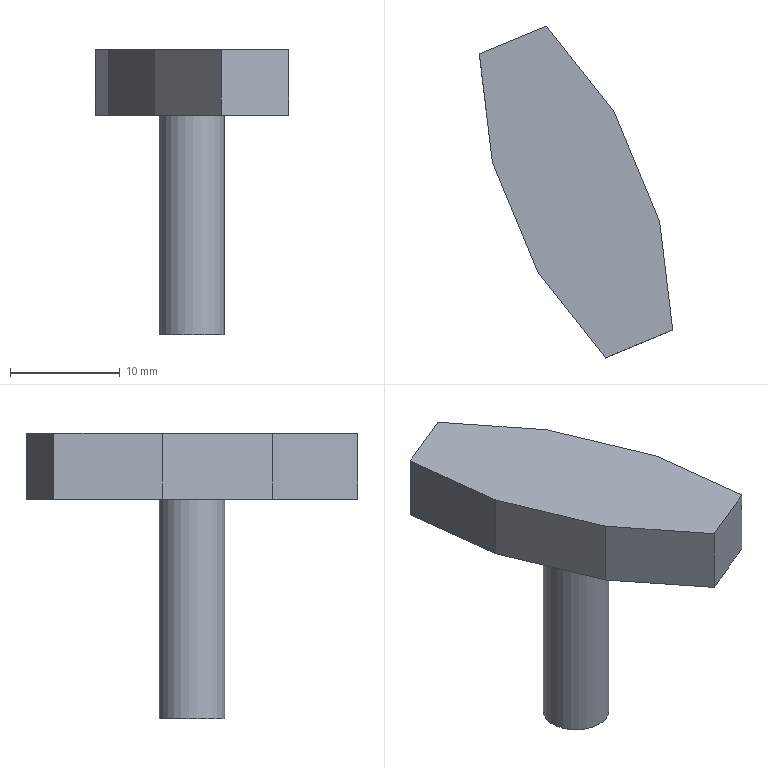Component | NX | MANUAL_SCREW | 1 solid | 12 faces | box 17.62 x 30.25 x 26 mm | volume 2418 mm3 | plane 11 | cylinder 1 | commonest cylinder face diameters 6 x1
STEP:
#1=CARTESIAN_POINT('',(0.,0.,0.));
#2=DIRECTION('',(0.,0.,1.));
#3=DIRECTION('',(1.,0.,0.));
#4=AXIS2_PLACEMENT_3D('',#1,#2,#3);
#5=CARTESIAN_POINT('',(97.911,100.613,38.296));
#6=VERTEX_POINT('',#5);
#7=CARTESIAN_POINT('',(96.724,110.478,38.296));
#8=VERTEX_POINT('',#7);
#9=CARTESIAN_POINT('',(97.911,100.613,38.296));
#10=DIRECTION('',(-0.1195,0.9928,0.));
#11=VECTOR('',#10,1.);
#12=LINE('',#9,#11);
#13=CARTESIAN_POINT('',(97.911,100.613,32.296));
#14=DIRECTION('',(0.9928,0.1195,0.));
#15=DIRECTION('',(0.1195,-0.9928,0.));
#16=AXIS2_PLACEMENT_3D('',#13,#14,#15);
#17=PLANE('',#16);
#18=CARTESIAN_POINT('',(0.,-6.));
#19=DIRECTION('',(-1.,0.));
#20=VECTOR('',#19,1.);
#21=LINE('',#18,#20);
#22=(GEOMETRIC_REPRESENTATION_CONTEXT(2)PARAMETRIC_REPRESENTATION_CONTEXT()REPRESENTATION_CONTEXT('',''));
#23=DEFINITIONAL_REPRESENTATION('',(#21),#22);
#24=PCURVE('',#17,#23);
#25=CARTESIAN_POINT('',(105.534,97.893,38.296));
#26=DIRECTION('',(0.,0.,-1.));
#27=DIRECTION('',(0.9237,0.383,0.));
#28=AXIS2_PLACEMENT_3D('',#25,#26,#27);
#29=PLANE('',#28);
#30=CARTESIAN_POINT('',(-6.,-5.433));
#31=DIRECTION('',(0.2699,-0.9629));
#32=VECTOR('',#31,1.);
#33=LINE('',#30,#32);
#34=(GEOMETRIC_REPRESENTATION_CONTEXT(2)PARAMETRIC_REPRESENTATION_CONTEXT()REPRESENTATION_CONTEXT('',''));
#35=DEFINITIONAL_REPRESENTATION('',(#33),#34);
#36=PCURVE('',#29,#35);
#37=SURFACE_CURVE('',#12,(#24,#36),.PCURVE_S1.);
#38=EDGE_CURVE('',#6,#8,#37,.T.);
#39=ORIENTED_EDGE('',*,*,#38,.T.);
#40=CARTESIAN_POINT('',(96.724,110.478,32.296));
#41=VERTEX_POINT('',#40);
#42=CARTESIAN_POINT('',(96.724,110.478,32.296));
#43=DIRECTION('',(0.,0.,1.));
#44=VECTOR('',#43,1.);
#45=LINE('',#42,#44);
#46=CARTESIAN_POINT('',(-9.936,0.));
#47=DIRECTION('',(0.,-1.));
#48=VECTOR('',#47,1.);
#49=LINE('',#46,#48);
#50=(GEOMETRIC_REPRESENTATION_CONTEXT(2)PARAMETRIC_REPRESENTATION_CONTEXT()REPRESENTATION_CONTEXT('',''));
#51=DEFINITIONAL_REPRESENTATION('',(#49),#50);
#52=PCURVE('',#17,#51);
#53=CARTESIAN_POINT('',(99.789,111.749,32.296));
#54=DIRECTION('',(0.383,-0.9237,0.));
#55=DIRECTION('',(0.,0.,-1.));
#56=AXIS2_PLACEMENT_3D('',#53,#54,#55);
#57=PLANE('',#56);
#58=CARTESIAN_POINT('',(0.,-3.318));
#59=DIRECTION('',(-1.,0.));
#60=VECTOR('',#59,1.);
#61=LINE('',#58,#60);
#62=(GEOMETRIC_REPRESENTATION_CONTEXT(2)PARAMETRIC_REPRESENTATION_CONTEXT()REPRESENTATION_CONTEXT('',''));
#63=DEFINITIONAL_REPRESENTATION('',(#61),#62);
#64=PCURVE('',#57,#63);
#65=SURFACE_CURVE('',#45,(#52,#64),.PCURVE_S1.);
#66=EDGE_CURVE('',#41,#8,#65,.T.);
#67=ORIENTED_EDGE('',*,*,#66,.F.);
#68=CARTESIAN_POINT('',(97.911,100.613,32.296));
#69=VERTEX_POINT('',#68);
#70=CARTESIAN_POINT('',(97.911,100.613,32.296));
#71=DIRECTION('',(-0.1195,0.9928,0.));
#72=VECTOR('',#71,1.);
#73=LINE('',#70,#72);
#74=CARTESIAN_POINT('',(0.,0.));
#75=DIRECTION('',(-1.,0.));
#76=VECTOR('',#75,1.);
#77=LINE('',#74,#76);
#78=(GEOMETRIC_REPRESENTATION_CONTEXT(2)PARAMETRIC_REPRESENTATION_CONTEXT()REPRESENTATION_CONTEXT('',''));
#79=DEFINITIONAL_REPRESENTATION('',(#77),#78);
#80=PCURVE('',#17,#79);
#81=CARTESIAN_POINT('',(105.534,97.893,32.296));
#82=DIRECTION('',(0.,0.,-1.));
#83=DIRECTION('',(0.9237,0.383,0.));
#84=AXIS2_PLACEMENT_3D('',#81,#82,#83);
#85=PLANE('',#84);
#86=CARTESIAN_POINT('',(-6.,-5.433));
#87=DIRECTION('',(0.2699,-0.9629));
#88=VECTOR('',#87,1.);
#89=LINE('',#86,#88);
#90=(GEOMETRIC_REPRESENTATION_CONTEXT(2)PARAMETRIC_REPRESENTATION_CONTEXT()REPRESENTATION_CONTEXT('',''));
#91=DEFINITIONAL_REPRESENTATION('',(#89),#90);
#92=PCURVE('',#85,#91);
#93=SURFACE_CURVE('',#73,(#80,#92),.PCURVE_S1.);
#94=EDGE_CURVE('',#69,#41,#93,.T.);
#95=ORIENTED_EDGE('',*,*,#94,.F.);
#96=CARTESIAN_POINT('',(97.911,100.613,32.296));
#97=DIRECTION('',(0.,0.,1.));
#98=VECTOR('',#97,1.);
#99=LINE('',#96,#98);
#100=CARTESIAN_POINT('',(0.,0.));
#101=DIRECTION('',(0.,-1.));
#102=VECTOR('',#101,1.);
#103=LINE('',#100,#102);
#104=(GEOMETRIC_REPRESENTATION_CONTEXT(2)PARAMETRIC_REPRESENTATION_CONTEXT()REPRESENTATION_CONTEXT('',''));
#105=DEFINITIONAL_REPRESENTATION('',(#103),#104);
#106=PCURVE('',#17,#105);
#107=CARTESIAN_POINT('',(102.073,90.576,32.296));
#108=DIRECTION('',(0.9237,0.383,0.));
#109=DIRECTION('',(0.383,-0.9237,0.));
#110=AXIS2_PLACEMENT_3D('',#107,#108,#109);
#111=PLANE('',#110);
#112=CARTESIAN_POINT('',(-10.866,0.));
#113=DIRECTION('',(0.,-1.));
#114=VECTOR('',#113,1.);
#115=LINE('',#112,#114);
#116=(GEOMETRIC_REPRESENTATION_CONTEXT(2)PARAMETRIC_REPRESENTATION_CONTEXT()REPRESENTATION_CONTEXT('',''));
#117=DEFINITIONAL_REPRESENTATION('',(#115),#116);
#118=PCURVE('',#111,#117);
#119=SURFACE_CURVE('',#99,(#106,#118),.PCURVE_S1.);
#120=EDGE_CURVE('',#69,#6,#119,.T.);
#121=ORIENTED_EDGE('',*,*,#120,.T.);
#122=EDGE_LOOP('',(#39,#67,#95,#121));
#123=FACE_BOUND('',#122,.T.);
#124=ADVANCED_FACE('',(#123),#17,.F.);
#125=CARTESIAN_POINT('',(102.854,113.02,38.296));
#126=VERTEX_POINT('',#125);
#127=CARTESIAN_POINT('',(99.789,111.749,38.296));
#128=DIRECTION('',(0.9237,0.383,0.));
#129=VECTOR('',#128,1.);
#130=LINE('',#127,#129);
#131=CARTESIAN_POINT('',(-6.,0.));
#132=DIRECTION('',(0.,1.));
#133=VECTOR('',#132,1.);
#134=LINE('',#131,#133);
#135=(GEOMETRIC_REPRESENTATION_CONTEXT(2)PARAMETRIC_REPRESENTATION_CONTEXT()REPRESENTATION_CONTEXT('',''));
#136=DEFINITIONAL_REPRESENTATION('',(#134),#135);
#137=PCURVE('',#57,#136);
#138=CARTESIAN_POINT('',(-0.,-15.));
#139=DIRECTION('',(1.,0.));
#140=VECTOR('',#139,1.);
#141=LINE('',#138,#140);
#142=(GEOMETRIC_REPRESENTATION_CONTEXT(2)PARAMETRIC_REPRESENTATION_CONTEXT()REPRESENTATION_CONTEXT('',''));
#143=DEFINITIONAL_REPRESENTATION('',(#141),#142);
#144=PCURVE('',#29,#143);
#145=SURFACE_CURVE('',#130,(#137,#144),.PCURVE_S1.);
#146=EDGE_CURVE('',#8,#126,#145,.T.);
#147=ORIENTED_EDGE('',*,*,#146,.T.);
#148=CARTESIAN_POINT('',(102.854,113.02,32.296));
#149=VERTEX_POINT('',#148);
#150=CARTESIAN_POINT('',(102.854,113.02,32.296));
#151=DIRECTION('',(0.,0.,1.));
#152=VECTOR('',#151,1.);
#153=LINE('',#150,#152);
#154=CARTESIAN_POINT('',(0.,3.318));
#155=DIRECTION('',(-1.,0.));
#156=VECTOR('',#155,1.);
#157=LINE('',#154,#156);
#158=(GEOMETRIC_REPRESENTATION_CONTEXT(2)PARAMETRIC_REPRESENTATION_CONTEXT()REPRESENTATION_CONTEXT('',''));
#159=DEFINITIONAL_REPRESENTATION('',(#157),#158);
#160=PCURVE('',#57,#159);
#161=CARTESIAN_POINT('',(102.854,113.02,32.296));
#162=DIRECTION('',(-0.786,-0.6182,0.));
#163=DIRECTION('',(-0.6182,0.786,0.));
#164=AXIS2_PLACEMENT_3D('',#161,#162,#163);
#165=PLANE('',#164);
#166=CARTESIAN_POINT('',(0.,0.));
#167=DIRECTION('',(0.,-1.));
#168=VECTOR('',#167,1.);
#169=LINE('',#166,#168);
#170=(GEOMETRIC_REPRESENTATION_CONTEXT(2)PARAMETRIC_REPRESENTATION_CONTEXT()REPRESENTATION_CONTEXT('',''));
#171=DEFINITIONAL_REPRESENTATION('',(#169),#170);
#172=PCURVE('',#165,#171);
#173=SURFACE_CURVE('',#153,(#160,#172),.PCURVE_S1.);
#174=EDGE_CURVE('',#149,#126,#173,.T.);
#175=ORIENTED_EDGE('',*,*,#174,.F.);
#176=CARTESIAN_POINT('',(96.724,110.478,32.296));
#177=DIRECTION('',(0.9237,0.383,0.));
#178=VECTOR('',#177,1.);
#179=LINE('',#176,#178);
#180=CARTESIAN_POINT('',(0.,-3.318));
#181=DIRECTION('',(0.,1.));
#182=VECTOR('',#181,1.);
#183=LINE('',#180,#182);
#184=(GEOMETRIC_REPRESENTATION_CONTEXT(2)PARAMETRIC_REPRESENTATION_CONTEXT()REPRESENTATION_CONTEXT('',''));
#185=DEFINITIONAL_REPRESENTATION('',(#183),#184);
#186=PCURVE('',#57,#185);
#187=CARTESIAN_POINT('',(-3.318,-15.));
#188=DIRECTION('',(1.,0.));
#189=VECTOR('',#188,1.);
#190=LINE('',#187,#189);
#191=(GEOMETRIC_REPRESENTATION_CONTEXT(2)PARAMETRIC_REPRESENTATION_CONTEXT()REPRESENTATION_CONTEXT('',''));
#192=DEFINITIONAL_REPRESENTATION('',(#190),#191);
#193=PCURVE('',#85,#192);
#194=SURFACE_CURVE('',#179,(#186,#193),.PCURVE_S1.);
#195=EDGE_CURVE('',#41,#149,#194,.T.);
#196=ORIENTED_EDGE('',*,*,#195,.F.);
#197=ORIENTED_EDGE('',*,*,#66,.T.);
#198=EDGE_LOOP('',(#147,#175,#196,#197));
#199=FACE_BOUND('',#198,.T.);
#200=ADVANCED_FACE('',(#199),#57,.F.);
#201=CARTESIAN_POINT('',(108.996,105.21,38.296));
#202=VERTEX_POINT('',#201);
#203=CARTESIAN_POINT('',(102.854,113.02,38.296));
#204=DIRECTION('',(0.6182,-0.786,0.));
#205=VECTOR('',#204,1.);
#206=LINE('',#203,#205);
#207=CARTESIAN_POINT('',(0.,-6.));
#208=DIRECTION('',(-1.,0.));
#209=VECTOR('',#208,1.);
#210=LINE('',#207,#209);
#211=(GEOMETRIC_REPRESENTATION_CONTEXT(2)PARAMETRIC_REPRESENTATION_CONTEXT()REPRESENTATION_CONTEXT('',''));
#212=DEFINITIONAL_REPRESENTATION('',(#210),#211);
#213=PCURVE('',#165,#212);
#214=CARTESIAN_POINT('',(3.318,-15.));
#215=DIRECTION('',(0.2699,0.9629));
#216=VECTOR('',#215,1.);
#217=LINE('',#214,#216);
#218=(GEOMETRIC_REPRESENTATION_CONTEXT(2)PARAMETRIC_REPRESENTATION_CONTEXT()REPRESENTATION_CONTEXT('',''));
#219=DEFINITIONAL_REPRESENTATION('',(#217),#218);
#220=PCURVE('',#29,#219);
#221=SURFACE_CURVE('',#206,(#213,#220),.PCURVE_S1.);
#222=EDGE_CURVE('',#126,#202,#221,.T.);
#223=ORIENTED_EDGE('',*,*,#222,.T.);
#224=CARTESIAN_POINT('',(108.996,105.21,32.296));
#225=VERTEX_POINT('',#224);
#226=CARTESIAN_POINT('',(108.996,105.21,32.296));
#227=DIRECTION('',(0.,0.,1.));
#228=VECTOR('',#227,1.);
#229=LINE('',#226,#228);
#230=CARTESIAN_POINT('',(-9.936,0.));
#231=DIRECTION('',(0.,-1.));
#232=VECTOR('',#231,1.);
#233=LINE('',#230,#232);
#234=(GEOMETRIC_REPRESENTATION_CONTEXT(2)PARAMETRIC_REPRESENTATION_CONTEXT()REPRESENTATION_CONTEXT('',''));
#235=DEFINITIONAL_REPRESENTATION('',(#233),#234);
#236=PCURVE('',#165,#235);
#237=CARTESIAN_POINT('',(111.077,100.191,32.296));
#238=DIRECTION('',(-0.9237,-0.383,0.));
#239=DIRECTION('',(-0.383,0.9237,0.));
#240=AXIS2_PLACEMENT_3D('',#237,#238,#239);
#241=PLANE('',#240);
#242=CARTESIAN_POINT('',(5.433,0.));
#243=DIRECTION('',(0.,-1.));
#244=VECTOR('',#243,1.);
#245=LINE('',#242,#244);
#246=(GEOMETRIC_REPRESENTATION_CONTEXT(2)PARAMETRIC_REPRESENTATION_CONTEXT()REPRESENTATION_CONTEXT('',''));
#247=DEFINITIONAL_REPRESENTATION('',(#245),#246);
#248=PCURVE('',#241,#247);
#249=SURFACE_CURVE('',#229,(#236,#248),.PCURVE_S1.);
#250=EDGE_CURVE('',#225,#202,#249,.T.);
#251=ORIENTED_EDGE('',*,*,#250,.F.);
#252=CARTESIAN_POINT('',(102.854,113.02,32.296));
#253=DIRECTION('',(0.6182,-0.786,0.));
#254=VECTOR('',#253,1.);
#255=LINE('',#252,#254);
#256=CARTESIAN_POINT('',(0.,0.));
#257=DIRECTION('',(-1.,0.));
#258=VECTOR('',#257,1.);
#259=LINE('',#256,#258);
#260=(GEOMETRIC_REPRESENTATION_CONTEXT(2)PARAMETRIC_REPRESENTATION_CONTEXT()REPRESENTATION_CONTEXT('',''));
#261=DEFINITIONAL_REPRESENTATION('',(#259),#260);
#262=PCURVE('',#165,#261);
#263=CARTESIAN_POINT('',(3.318,-15.));
#264=DIRECTION('',(0.2699,0.9629));
#265=VECTOR('',#264,1.);
#266=LINE('',#263,#265);
#267=(GEOMETRIC_REPRESENTATION_CONTEXT(2)PARAMETRIC_REPRESENTATION_CONTEXT()REPRESENTATION_CONTEXT('',''));
#268=DEFINITIONAL_REPRESENTATION('',(#266),#267);
#269=PCURVE('',#85,#268);
#270=SURFACE_CURVE('',#255,(#262,#269),.PCURVE_S1.);
#271=EDGE_CURVE('',#149,#225,#270,.T.);
#272=ORIENTED_EDGE('',*,*,#271,.F.);
#273=ORIENTED_EDGE('',*,*,#174,.T.);
#274=EDGE_LOOP('',(#223,#251,#272,#273));
#275=FACE_BOUND('',#274,.T.);
#276=ADVANCED_FACE('',(#275),#165,.F.);
#277=CARTESIAN_POINT('',(113.158,95.172,38.296));
#278=VERTEX_POINT('',#277);
#279=CARTESIAN_POINT('',(111.077,100.191,38.296));
#280=DIRECTION('',(0.383,-0.9237,0.));
#281=VECTOR('',#280,1.);
#282=LINE('',#279,#281);
#283=CARTESIAN_POINT('',(0.,-6.));
#284=DIRECTION('',(-1.,0.));
#285=VECTOR('',#284,1.);
#286=LINE('',#283,#285);
#287=(GEOMETRIC_REPRESENTATION_CONTEXT(2)PARAMETRIC_REPRESENTATION_CONTEXT()REPRESENTATION_CONTEXT('',''));
#288=DEFINITIONAL_REPRESENTATION('',(#286),#287);
#289=PCURVE('',#241,#288);
#290=CARTESIAN_POINT('',(6.,-0.));
#291=DIRECTION('',(0.,1.));
#292=VECTOR('',#291,1.);
#293=LINE('',#290,#292);
#294=(GEOMETRIC_REPRESENTATION_CONTEXT(2)PARAMETRIC_REPRESENTATION_CONTEXT()REPRESENTATION_CONTEXT('',''));
#295=DEFINITIONAL_REPRESENTATION('',(#293),#294);
#296=PCURVE('',#29,#295);
#297=SURFACE_CURVE('',#282,(#289,#296),.PCURVE_S1.);
#298=EDGE_CURVE('',#202,#278,#297,.T.);
#299=ORIENTED_EDGE('',*,*,#298,.T.);
#300=CARTESIAN_POINT('',(113.158,95.172,32.296));
#301=VERTEX_POINT('',#300);
#302=CARTESIAN_POINT('',(113.158,95.172,32.296));
#303=DIRECTION('',(0.,0.,1.));
#304=VECTOR('',#303,1.);
#305=LINE('',#302,#304);
#306=CARTESIAN_POINT('',(-5.433,0.));
#307=DIRECTION('',(0.,-1.));
#308=VECTOR('',#307,1.);
#309=LINE('',#306,#308);
#310=(GEOMETRIC_REPRESENTATION_CONTEXT(2)PARAMETRIC_REPRESENTATION_CONTEXT()REPRESENTATION_CONTEXT('',''));
#311=DEFINITIONAL_REPRESENTATION('',(#309),#310);
#312=PCURVE('',#241,#311);
#313=CARTESIAN_POINT('',(113.158,95.172,32.296));
#314=DIRECTION('',(-0.9928,-0.1195,0.));
#315=DIRECTION('',(-0.1195,0.9928,0.));
#316=AXIS2_PLACEMENT_3D('',#313,#314,#315);
#317=PLANE('',#316);
#318=CARTESIAN_POINT('',(0.,0.));
#319=DIRECTION('',(0.,-1.));
#320=VECTOR('',#319,1.);
#321=LINE('',#318,#320);
#322=(GEOMETRIC_REPRESENTATION_CONTEXT(2)PARAMETRIC_REPRESENTATION_CONTEXT()REPRESENTATION_CONTEXT('',''));
#323=DEFINITIONAL_REPRESENTATION('',(#321),#322);
#324=PCURVE('',#317,#323);
#325=SURFACE_CURVE('',#305,(#312,#324),.PCURVE_S1.);
#326=EDGE_CURVE('',#301,#278,#325,.T.);
#327=ORIENTED_EDGE('',*,*,#326,.F.);
#328=CARTESIAN_POINT('',(108.996,105.21,32.296));
#329=DIRECTION('',(0.383,-0.9237,0.));
#330=VECTOR('',#329,1.);
#331=LINE('',#328,#330);
#332=CARTESIAN_POINT('',(5.433,0.));
#333=DIRECTION('',(-1.,0.));
#334=VECTOR('',#333,1.);
#335=LINE('',#332,#334);
#336=(GEOMETRIC_REPRESENTATION_CONTEXT(2)PARAMETRIC_REPRESENTATION_CONTEXT()REPRESENTATION_CONTEXT('',''));
#337=DEFINITIONAL_REPRESENTATION('',(#335),#336);
#338=PCURVE('',#241,#337);
#339=CARTESIAN_POINT('',(6.,-5.433));
#340=DIRECTION('',(-0.,1.));
#341=VECTOR('',#340,1.);
#342=LINE('',#339,#341);
#343=(GEOMETRIC_REPRESENTATION_CONTEXT(2)PARAMETRIC_REPRESENTATION_CONTEXT()REPRESENTATION_CONTEXT('',''));
#344=DEFINITIONAL_REPRESENTATION('',(#342),#343);
#345=PCURVE('',#85,#344);
#346=SURFACE_CURVE('',#331,(#338,#345),.PCURVE_S1.);
#347=EDGE_CURVE('',#225,#301,#346,.T.);
#348=ORIENTED_EDGE('',*,*,#347,.F.);
#349=ORIENTED_EDGE('',*,*,#250,.T.);
#350=EDGE_LOOP('',(#299,#327,#348,#349));
#351=FACE_BOUND('',#350,.T.);
#352=ADVANCED_FACE('',(#351),#241,.F.);
#353=CARTESIAN_POINT('',(114.345,85.308,38.296));
#354=VERTEX_POINT('',#353);
#355=CARTESIAN_POINT('',(113.158,95.172,38.296));
#356=DIRECTION('',(0.1195,-0.9928,0.));
#357=VECTOR('',#356,1.);
#358=LINE('',#355,#357);
#359=CARTESIAN_POINT('',(0.,-6.));
#360=DIRECTION('',(-1.,0.));
#361=VECTOR('',#360,1.);
#362=LINE('',#359,#361);
#363=(GEOMETRIC_REPRESENTATION_CONTEXT(2)PARAMETRIC_REPRESENTATION_CONTEXT()REPRESENTATION_CONTEXT('',''));
#364=DEFINITIONAL_REPRESENTATION('',(#362),#363);
#365=PCURVE('',#317,#364);
#366=CARTESIAN_POINT('',(6.,5.433));
#367=DIRECTION('',(-0.2699,0.9629));
#368=VECTOR('',#367,1.);
#369=LINE('',#366,#368);
#370=(GEOMETRIC_REPRESENTATION_CONTEXT(2)PARAMETRIC_REPRESENTATION_CONTEXT()REPRESENTATION_CONTEXT('',''));
#371=DEFINITIONAL_REPRESENTATION('',(#369),#370);
#372=PCURVE('',#29,#371);
#373=SURFACE_CURVE('',#358,(#365,#372),.PCURVE_S1.);
#374=EDGE_CURVE('',#278,#354,#373,.T.);
#375=ORIENTED_EDGE('',*,*,#374,.T.);
#376=CARTESIAN_POINT('',(114.345,85.308,32.296));
#377=VERTEX_POINT('',#376);
#378=CARTESIAN_POINT('',(114.345,85.308,32.296));
#379=DIRECTION('',(0.,0.,1.));
#380=VECTOR('',#379,1.);
#381=LINE('',#378,#380);
#382=CARTESIAN_POINT('',(-9.936,0.));
#383=DIRECTION('',(0.,-1.));
#384=VECTOR('',#383,1.);
#385=LINE('',#382,#384);
#386=(GEOMETRIC_REPRESENTATION_CONTEXT(2)PARAMETRIC_REPRESENTATION_CONTEXT()REPRESENTATION_CONTEXT('',''));
#387=DEFINITIONAL_REPRESENTATION('',(#385),#386);
#388=PCURVE('',#317,#387);
#389=CARTESIAN_POINT('',(111.28,84.037,32.296));
#390=DIRECTION('',(-0.383,0.9237,0.));
#391=DIRECTION('',(0.,0.,1.));
#392=AXIS2_PLACEMENT_3D('',#389,#390,#391);
#393=PLANE('',#392);
#394=CARTESIAN_POINT('',(0.,3.318));
#395=DIRECTION('',(1.,0.));
#396=VECTOR('',#395,1.);
#397=LINE('',#394,#396);
#398=(GEOMETRIC_REPRESENTATION_CONTEXT(2)PARAMETRIC_REPRESENTATION_CONTEXT()REPRESENTATION_CONTEXT('',''));
#399=DEFINITIONAL_REPRESENTATION('',(#397),#398);
#400=PCURVE('',#393,#399);
#401=SURFACE_CURVE('',#381,(#388,#400),.PCURVE_S1.);
#402=EDGE_CURVE('',#377,#354,#401,.T.);
#403=ORIENTED_EDGE('',*,*,#402,.F.);
#404=CARTESIAN_POINT('',(113.158,95.172,32.296));
#405=DIRECTION('',(0.1195,-0.9928,0.));
#406=VECTOR('',#405,1.);
#407=LINE('',#404,#406);
#408=CARTESIAN_POINT('',(0.,0.));
#409=DIRECTION('',(-1.,0.));
#410=VECTOR('',#409,1.);
#411=LINE('',#408,#410);
#412=(GEOMETRIC_REPRESENTATION_CONTEXT(2)PARAMETRIC_REPRESENTATION_CONTEXT()REPRESENTATION_CONTEXT('',''));
#413=DEFINITIONAL_REPRESENTATION('',(#411),#412);
#414=PCURVE('',#317,#413);
#415=CARTESIAN_POINT('',(6.,5.433));
#416=DIRECTION('',(-0.2699,0.9629));
#417=VECTOR('',#416,1.);
#418=LINE('',#415,#417);
#419=(GEOMETRIC_REPRESENTATION_CONTEXT(2)PARAMETRIC_REPRESENTATION_CONTEXT()REPRESENTATION_CONTEXT('',''));
#420=DEFINITIONAL_REPRESENTATION('',(#418),#419);
#421=PCURVE('',#85,#420);
#422=SURFACE_CURVE('',#407,(#414,#421),.PCURVE_S1.);
#423=EDGE_CURVE('',#301,#377,#422,.T.);
#424=ORIENTED_EDGE('',*,*,#423,.F.);
#425=ORIENTED_EDGE('',*,*,#326,.T.);
#426=EDGE_LOOP('',(#375,#403,#424,#425));
#427=FACE_BOUND('',#426,.T.);
#428=ADVANCED_FACE('',(#427),#317,.F.);
#429=CARTESIAN_POINT('',(108.215,82.766,38.296));
#430=VERTEX_POINT('',#429);
#431=CARTESIAN_POINT('',(111.28,84.037,38.296));
#432=DIRECTION('',(-0.9237,-0.383,0.));
#433=VECTOR('',#432,1.);
#434=LINE('',#431,#433);
#435=CARTESIAN_POINT('',(6.,0.));
#436=DIRECTION('',(0.,-1.));
#437=VECTOR('',#436,1.);
#438=LINE('',#435,#437);
#439=(GEOMETRIC_REPRESENTATION_CONTEXT(2)PARAMETRIC_REPRESENTATION_CONTEXT()REPRESENTATION_CONTEXT('',''));
#440=DEFINITIONAL_REPRESENTATION('',(#438),#439);
#441=PCURVE('',#393,#440);
#442=CARTESIAN_POINT('',(-0.,15.));
#443=DIRECTION('',(-1.,0.));
#444=VECTOR('',#443,1.);
#445=LINE('',#442,#444);
#446=(GEOMETRIC_REPRESENTATION_CONTEXT(2)PARAMETRIC_REPRESENTATION_CONTEXT()REPRESENTATION_CONTEXT('',''));
#447=DEFINITIONAL_REPRESENTATION('',(#445),#446);
#448=PCURVE('',#29,#447);
#449=SURFACE_CURVE('',#434,(#441,#448),.PCURVE_S1.);
#450=EDGE_CURVE('',#354,#430,#449,.T.);
#451=ORIENTED_EDGE('',*,*,#450,.T.);
#452=CARTESIAN_POINT('',(108.215,82.766,32.296));
#453=VERTEX_POINT('',#452);
#454=CARTESIAN_POINT('',(108.215,82.766,32.296));
#455=DIRECTION('',(0.,0.,1.));
#456=VECTOR('',#455,1.);
#457=LINE('',#454,#456);
#458=CARTESIAN_POINT('',(0.,-3.318));
#459=DIRECTION('',(1.,0.));
#460=VECTOR('',#459,1.);
#461=LINE('',#458,#460);
#462=(GEOMETRIC_REPRESENTATION_CONTEXT(2)PARAMETRIC_REPRESENTATION_CONTEXT()REPRESENTATION_CONTEXT('',''));
#463=DEFINITIONAL_REPRESENTATION('',(#461),#462);
#464=PCURVE('',#393,#463);
#465=CARTESIAN_POINT('',(108.215,82.766,32.296));
#466=DIRECTION('',(0.786,0.6182,0.));
#467=DIRECTION('',(0.6182,-0.786,0.));
#468=AXIS2_PLACEMENT_3D('',#465,#466,#467);
#469=PLANE('',#468);
#470=CARTESIAN_POINT('',(0.,0.));
#471=DIRECTION('',(0.,-1.));
#472=VECTOR('',#471,1.);
#473=LINE('',#470,#472);
#474=(GEOMETRIC_REPRESENTATION_CONTEXT(2)PARAMETRIC_REPRESENTATION_CONTEXT()REPRESENTATION_CONTEXT('',''));
#475=DEFINITIONAL_REPRESENTATION('',(#473),#474);
#476=PCURVE('',#469,#475);
#477=SURFACE_CURVE('',#457,(#464,#476),.PCURVE_S1.);
#478=EDGE_CURVE('',#453,#430,#477,.T.);
#479=ORIENTED_EDGE('',*,*,#478,.F.);
#480=CARTESIAN_POINT('',(114.345,85.308,32.296));
#481=DIRECTION('',(-0.9237,-0.383,0.));
#482=VECTOR('',#481,1.);
#483=LINE('',#480,#482);
#484=CARTESIAN_POINT('',(0.,3.318));
#485=DIRECTION('',(0.,-1.));
#486=VECTOR('',#485,1.);
#487=LINE('',#484,#486);
#488=(GEOMETRIC_REPRESENTATION_CONTEXT(2)PARAMETRIC_REPRESENTATION_CONTEXT()REPRESENTATION_CONTEXT('',''));
#489=DEFINITIONAL_REPRESENTATION('',(#487),#488);
#490=PCURVE('',#393,#489);
#491=CARTESIAN_POINT('',(3.318,15.));
#492=DIRECTION('',(-1.,0.));
#493=VECTOR('',#492,1.);
#494=LINE('',#491,#493);
#495=(GEOMETRIC_REPRESENTATION_CONTEXT(2)PARAMETRIC_REPRESENTATION_CONTEXT()REPRESENTATION_CONTEXT('',''));
#496=DEFINITIONAL_REPRESENTATION('',(#494),#495);
#497=PCURVE('',#85,#496);
#498=SURFACE_CURVE('',#483,(#490,#497),.PCURVE_S1.);
#499=EDGE_CURVE('',#377,#453,#498,.T.);
#500=ORIENTED_EDGE('',*,*,#499,.F.);
#501=ORIENTED_EDGE('',*,*,#402,.T.);
#502=EDGE_LOOP('',(#451,#479,#500,#501));
#503=FACE_BOUND('',#502,.T.);
#504=ADVANCED_FACE('',(#503),#393,.F.);
#505=CARTESIAN_POINT('',(102.073,90.576,38.296));
#506=VERTEX_POINT('',#505);
#507=CARTESIAN_POINT('',(108.215,82.766,38.296));
#508=DIRECTION('',(-0.6182,0.786,0.));
#509=VECTOR('',#508,1.);
#510=LINE('',#507,#509);
#511=CARTESIAN_POINT('',(0.,-6.));
#512=DIRECTION('',(-1.,0.));
#513=VECTOR('',#512,1.);
#514=LINE('',#511,#513);
#515=(GEOMETRIC_REPRESENTATION_CONTEXT(2)PARAMETRIC_REPRESENTATION_CONTEXT()REPRESENTATION_CONTEXT('',''));
#516=DEFINITIONAL_REPRESENTATION('',(#514),#515);
#517=PCURVE('',#469,#516);
#518=CARTESIAN_POINT('',(-3.318,15.));
#519=DIRECTION('',(-0.2699,-0.9629));
#520=VECTOR('',#519,1.);
#521=LINE('',#518,#520);
#522=(GEOMETRIC_REPRESENTATION_CONTEXT(2)PARAMETRIC_REPRESENTATION_CONTEXT()REPRESENTATION_CONTEXT('',''));
#523=DEFINITIONAL_REPRESENTATION('',(#521),#522);
#524=PCURVE('',#29,#523);
#525=SURFACE_CURVE('',#510,(#517,#524),.PCURVE_S1.);
#526=EDGE_CURVE('',#430,#506,#525,.T.);
#527=ORIENTED_EDGE('',*,*,#526,.T.);
#528=CARTESIAN_POINT('',(102.073,90.576,32.296));
#529=VERTEX_POINT('',#528);
#530=CARTESIAN_POINT('',(102.073,90.576,32.296));
#531=DIRECTION('',(0.,0.,1.));
#532=VECTOR('',#531,1.);
#533=LINE('',#530,#532);
#534=CARTESIAN_POINT('',(-9.936,0.));
#535=DIRECTION('',(0.,-1.));
#536=VECTOR('',#535,1.);
#537=LINE('',#534,#536);
#538=(GEOMETRIC_REPRESENTATION_CONTEXT(2)PARAMETRIC_REPRESENTATION_CONTEXT()REPRESENTATION_CONTEXT('',''));
#539=DEFINITIONAL_REPRESENTATION('',(#537),#538);
#540=PCURVE('',#469,#539);
#541=CARTESIAN_POINT('',(0.,0.));
#542=DIRECTION('',(0.,-1.));
#543=VECTOR('',#542,1.);
#544=LINE('',#541,#543);
#545=(GEOMETRIC_REPRESENTATION_CONTEXT(2)PARAMETRIC_REPRESENTATION_CONTEXT()REPRESENTATION_CONTEXT('',''));
#546=DEFINITIONAL_REPRESENTATION('',(#544),#545);
#547=PCURVE('',#111,#546);
#548=SURFACE_CURVE('',#533,(#540,#547),.PCURVE_S1.);
#549=EDGE_CURVE('',#529,#506,#548,.T.);
#550=ORIENTED_EDGE('',*,*,#549,.F.);
#551=CARTESIAN_POINT('',(108.215,82.766,32.296));
#552=DIRECTION('',(-0.6182,0.786,0.));
#553=VECTOR('',#552,1.);
#554=LINE('',#551,#553);
#555=CARTESIAN_POINT('',(0.,0.));
#556=DIRECTION('',(-1.,0.));
#557=VECTOR('',#556,1.);
#558=LINE('',#555,#557);
#559=(GEOMETRIC_REPRESENTATION_CONTEXT(2)PARAMETRIC_REPRESENTATION_CONTEXT()REPRESENTATION_CONTEXT('',''));
#560=DEFINITIONAL_REPRESENTATION('',(#558),#559);
#561=PCURVE('',#469,#560);
#562=CARTESIAN_POINT('',(-3.318,15.));
#563=DIRECTION('',(-0.2699,-0.9629));
#564=VECTOR('',#563,1.);
#565=LINE('',#562,#564);
#566=(GEOMETRIC_REPRESENTATION_CONTEXT(2)PARAMETRIC_REPRESENTATION_CONTEXT()REPRESENTATION_CONTEXT('',''));
#567=DEFINITIONAL_REPRESENTATION('',(#565),#566);
#568=PCURVE('',#85,#567);
#569=SURFACE_CURVE('',#554,(#561,#568),.PCURVE_S1.);
#570=EDGE_CURVE('',#453,#529,#569,.T.);
#571=ORIENTED_EDGE('',*,*,#570,.F.);
#572=ORIENTED_EDGE('',*,*,#478,.T.);
#573=EDGE_LOOP('',(#527,#550,#571,#572));
#574=FACE_BOUND('',#573,.T.);
#575=ADVANCED_FACE('',(#574),#469,.F.);
#576=CARTESIAN_POINT('',(102.073,90.576,38.296));
#577=DIRECTION('',(-0.383,0.9237,0.));
#578=VECTOR('',#577,1.);
#579=LINE('',#576,#578);
#580=CARTESIAN_POINT('',(0.,-6.));
#581=DIRECTION('',(-1.,0.));
#582=VECTOR('',#581,1.);
#583=LINE('',#580,#582);
#584=(GEOMETRIC_REPRESENTATION_CONTEXT(2)PARAMETRIC_REPRESENTATION_CONTEXT()REPRESENTATION_CONTEXT('',''));
#585=DEFINITIONAL_REPRESENTATION('',(#583),#584);
#586=PCURVE('',#111,#585);
#587=CARTESIAN_POINT('',(-6.,5.433));
#588=DIRECTION('',(0.,-1.));
#589=VECTOR('',#588,1.);
#590=LINE('',#587,#589);
#591=(GEOMETRIC_REPRESENTATION_CONTEXT(2)PARAMETRIC_REPRESENTATION_CONTEXT()REPRESENTATION_CONTEXT('',''));
#592=DEFINITIONAL_REPRESENTATION('',(#590),#591);
#593=PCURVE('',#29,#592);
#594=SURFACE_CURVE('',#579,(#586,#593),.PCURVE_S1.);
#595=EDGE_CURVE('',#506,#6,#594,.T.);
#596=ORIENTED_EDGE('',*,*,#595,.T.);
#597=ORIENTED_EDGE('',*,*,#120,.F.);
#598=CARTESIAN_POINT('',(99.992,95.595,32.296));
#599=DIRECTION('',(-0.383,0.9237,0.));
#600=VECTOR('',#599,1.);
#601=LINE('',#598,#600);
#602=CARTESIAN_POINT('',(-5.433,0.));
#603=DIRECTION('',(-1.,0.));
#604=VECTOR('',#603,1.);
#605=LINE('',#602,#604);
#606=(GEOMETRIC_REPRESENTATION_CONTEXT(2)PARAMETRIC_REPRESENTATION_CONTEXT()REPRESENTATION_CONTEXT('',''));
#607=DEFINITIONAL_REPRESENTATION('',(#605),#606);
#608=PCURVE('',#111,#607);
#609=CARTESIAN_POINT('',(-6.,-0.));
#610=DIRECTION('',(0.,-1.));
#611=VECTOR('',#610,1.);
#612=LINE('',#609,#611);
#613=(GEOMETRIC_REPRESENTATION_CONTEXT(2)PARAMETRIC_REPRESENTATION_CONTEXT()REPRESENTATION_CONTEXT('',''));
#614=DEFINITIONAL_REPRESENTATION('',(#612),#613);
#615=PCURVE('',#85,#614);
#616=SURFACE_CURVE('',#601,(#608,#615),.PCURVE_S1.);
#617=EDGE_CURVE('',#529,#69,#616,.T.);
#618=ORIENTED_EDGE('',*,*,#617,.F.);
#619=ORIENTED_EDGE('',*,*,#549,.T.);
#620=EDGE_LOOP('',(#596,#597,#618,#619));
#621=FACE_BOUND('',#620,.T.);
#622=ADVANCED_FACE('',(#621),#111,.F.);
#623=CARTESIAN_POINT('',(108.306,99.042,32.296));
#624=VERTEX_POINT('',#623);
#625=CARTESIAN_POINT('',(105.534,97.893,32.296));
#626=DIRECTION('',(0.,0.,-1.));
#627=DIRECTION('',(0.9237,0.383,0.));
#628=AXIS2_PLACEMENT_3D('',#625,#626,#627);
#629=CIRCLE('',#628,3.);
#630=CARTESIAN_POINT('',(0.,0.));
#631=DIRECTION('',(1.,0.));
#632=AXIS2_PLACEMENT_2D('',#630,#631);
#633=CIRCLE('',#632,3.);
#634=(GEOMETRIC_REPRESENTATION_CONTEXT(2)PARAMETRIC_REPRESENTATION_CONTEXT()REPRESENTATION_CONTEXT('',''));
#635=DEFINITIONAL_REPRESENTATION('',(#633),#634);
#636=PCURVE('',#85,#635);
#637=CARTESIAN_POINT('',(105.534,97.893,12.296));
#638=DIRECTION('',(0.,0.,1.));
#639=DIRECTION('',(-0.9237,-0.383,0.));
#640=AXIS2_PLACEMENT_3D('',#637,#638,#639);
#641=CYLINDRICAL_SURFACE('',#640,3.);
#642=CARTESIAN_POINT('',(9.425,20.));
#643=DIRECTION('',(-1.,0.));
#644=VECTOR('',#643,1.);
#645=LINE('',#642,#644);
#646=(GEOMETRIC_REPRESENTATION_CONTEXT(2)PARAMETRIC_REPRESENTATION_CONTEXT()REPRESENTATION_CONTEXT('',''));
#647=DEFINITIONAL_REPRESENTATION('',(#645),#646);
#648=PCURVE('',#641,#647);
#649=SURFACE_CURVE('',#629,(#636,#648),.PCURVE_S1.);
#650=EDGE_CURVE('',#624,#624,#649,.T.);
#651=ORIENTED_EDGE('',*,*,#650,.F.);
#652=EDGE_LOOP('',(#651));
#653=FACE_BOUND('',#652,.T.);
#654=ORIENTED_EDGE('',*,*,#617,.T.);
#655=ORIENTED_EDGE('',*,*,#94,.T.);
#656=ORIENTED_EDGE('',*,*,#195,.T.);
#657=ORIENTED_EDGE('',*,*,#271,.T.);
#658=ORIENTED_EDGE('',*,*,#347,.T.);
#659=ORIENTED_EDGE('',*,*,#423,.T.);
#660=ORIENTED_EDGE('',*,*,#499,.T.);
#661=ORIENTED_EDGE('',*,*,#570,.T.);
#662=EDGE_LOOP('',(#654,#655,#656,#657,#658,#659,#660,#661));
#663=FACE_BOUND('',#662,.T.);
#664=ADVANCED_FACE('',(#653,#663),#85,.T.);
#665=ORIENTED_EDGE('',*,*,#38,.F.);
#666=ORIENTED_EDGE('',*,*,#595,.F.);
#667=ORIENTED_EDGE('',*,*,#526,.F.);
#668=ORIENTED_EDGE('',*,*,#450,.F.);
#669=ORIENTED_EDGE('',*,*,#374,.F.);
#670=ORIENTED_EDGE('',*,*,#298,.F.);
#671=ORIENTED_EDGE('',*,*,#222,.F.);
#672=ORIENTED_EDGE('',*,*,#146,.F.);
#673=EDGE_LOOP('',(#665,#666,#667,#668,#669,#670,#671,#672));
#674=FACE_BOUND('',#673,.T.);
#675=ADVANCED_FACE('',(#674),#29,.F.);
#676=CARTESIAN_POINT('',(108.306,99.042,12.296));
#677=VERTEX_POINT('',#676);
#678=CARTESIAN_POINT('',(105.534,97.893,12.296));
#679=DIRECTION('',(0.,0.,-1.));
#680=DIRECTION('',(0.9237,0.383,0.));
#681=AXIS2_PLACEMENT_3D('',#678,#679,#680);
#682=CIRCLE('',#681,3.);
#683=CARTESIAN_POINT('',(9.425,0.));
#684=DIRECTION('',(-1.,0.));
#685=VECTOR('',#684,1.);
#686=LINE('',#683,#685);
#687=(GEOMETRIC_REPRESENTATION_CONTEXT(2)PARAMETRIC_REPRESENTATION_CONTEXT()REPRESENTATION_CONTEXT('',''));
#688=DEFINITIONAL_REPRESENTATION('',(#686),#687);
#689=PCURVE('',#641,#688);
#690=CARTESIAN_POINT('',(105.534,97.893,12.296));
#691=DIRECTION('',(0.,0.,-1.));
#692=DIRECTION('',(0.9237,0.383,0.));
#693=AXIS2_PLACEMENT_3D('',#690,#691,#692);
#694=PLANE('',#693);
#695=CARTESIAN_POINT('',(0.,0.));
#696=DIRECTION('',(1.,0.));
#697=AXIS2_PLACEMENT_2D('',#695,#696);
#698=CIRCLE('',#697,3.);
#699=(GEOMETRIC_REPRESENTATION_CONTEXT(2)PARAMETRIC_REPRESENTATION_CONTEXT()REPRESENTATION_CONTEXT('',''));
#700=DEFINITIONAL_REPRESENTATION('',(#698),#699);
#701=PCURVE('',#694,#700);
#702=SURFACE_CURVE('',#682,(#689,#701),.PCURVE_S1.);
#703=EDGE_CURVE('',#677,#677,#702,.T.);
#704=ORIENTED_EDGE('',*,*,#703,.F.);
#705=CARTESIAN_POINT('',(108.306,99.042,12.296));
#706=CARTESIAN_POINT('',(108.306,99.042,32.296));
#707=B_SPLINE_CURVE_WITH_KNOTS('',1,(#705,#706),.UNSPECIFIED.,.F.,.F.,(2,2),(0.,20.),.PIECEWISE_BEZIER_KNOTS.);
#708=CARTESIAN_POINT('',(9.425,0.));
#709=DIRECTION('',(0.,1.));
#710=VECTOR('',#709,1.);
#711=LINE('',#708,#710);
#712=(GEOMETRIC_REPRESENTATION_CONTEXT(2)PARAMETRIC_REPRESENTATION_CONTEXT()REPRESENTATION_CONTEXT('',''));
#713=DEFINITIONAL_REPRESENTATION('',(#711),#712);
#714=PCURVE('',#641,#713);
#715=CARTESIAN_POINT('',(3.142,0.));
#716=DIRECTION('',(0.,1.));
#717=VECTOR('',#716,1.);
#718=LINE('',#715,#717);
#719=(GEOMETRIC_REPRESENTATION_CONTEXT(2)PARAMETRIC_REPRESENTATION_CONTEXT()REPRESENTATION_CONTEXT('',''));
#720=DEFINITIONAL_REPRESENTATION('',(#718),#719);
#721=PCURVE('',#641,#720);
#722=SEAM_CURVE('',#707,(#714,#721),.PCURVE_S1.);
#723=EDGE_CURVE('',#677,#624,#722,.T.);
#724=ORIENTED_EDGE('',*,*,#723,.T.);
#725=ORIENTED_EDGE('',*,*,#650,.T.);
#726=ORIENTED_EDGE('',*,*,#723,.F.);
#727=EDGE_LOOP('',(#704,#724,#725,#726));
#728=FACE_BOUND('',#727,.T.);
#729=ADVANCED_FACE('',(#728),#641,.T.);
#730=ORIENTED_EDGE('',*,*,#703,.T.);
#731=EDGE_LOOP('',(#730));
#732=FACE_BOUND('',#731,.T.);
#733=ADVANCED_FACE('',(#732),#694,.T.);
#734=CLOSED_SHELL('',(#124,#200,#276,#352,#428,#504,#575,#622,#664,#675,#729,#733));
#735=MANIFOLD_SOLID_BREP('',#734);
#736=(LENGTH_UNIT()NAMED_UNIT(*)SI_UNIT(.MILLI.,.METRE.));
#737=UNCERTAINTY_MEASURE_WITH_UNIT(LENGTH_MEASURE(0.000001),#736,'','');
#738=(NAMED_UNIT(*)PLANE_ANGLE_UNIT()SI_UNIT($,.RADIAN.));
#739=(NAMED_UNIT(*)SI_UNIT($,.STERADIAN.)SOLID_ANGLE_UNIT());
#740=(GEOMETRIC_REPRESENTATION_CONTEXT(3)GLOBAL_UNCERTAINTY_ASSIGNED_CONTEXT((#737))GLOBAL_UNIT_ASSIGNED_CONTEXT((#736,#738,#739))REPRESENTATION_CONTEXT('',''));
#741=ADVANCED_BREP_SHAPE_REPRESENTATION('',(#4,#735),#740);